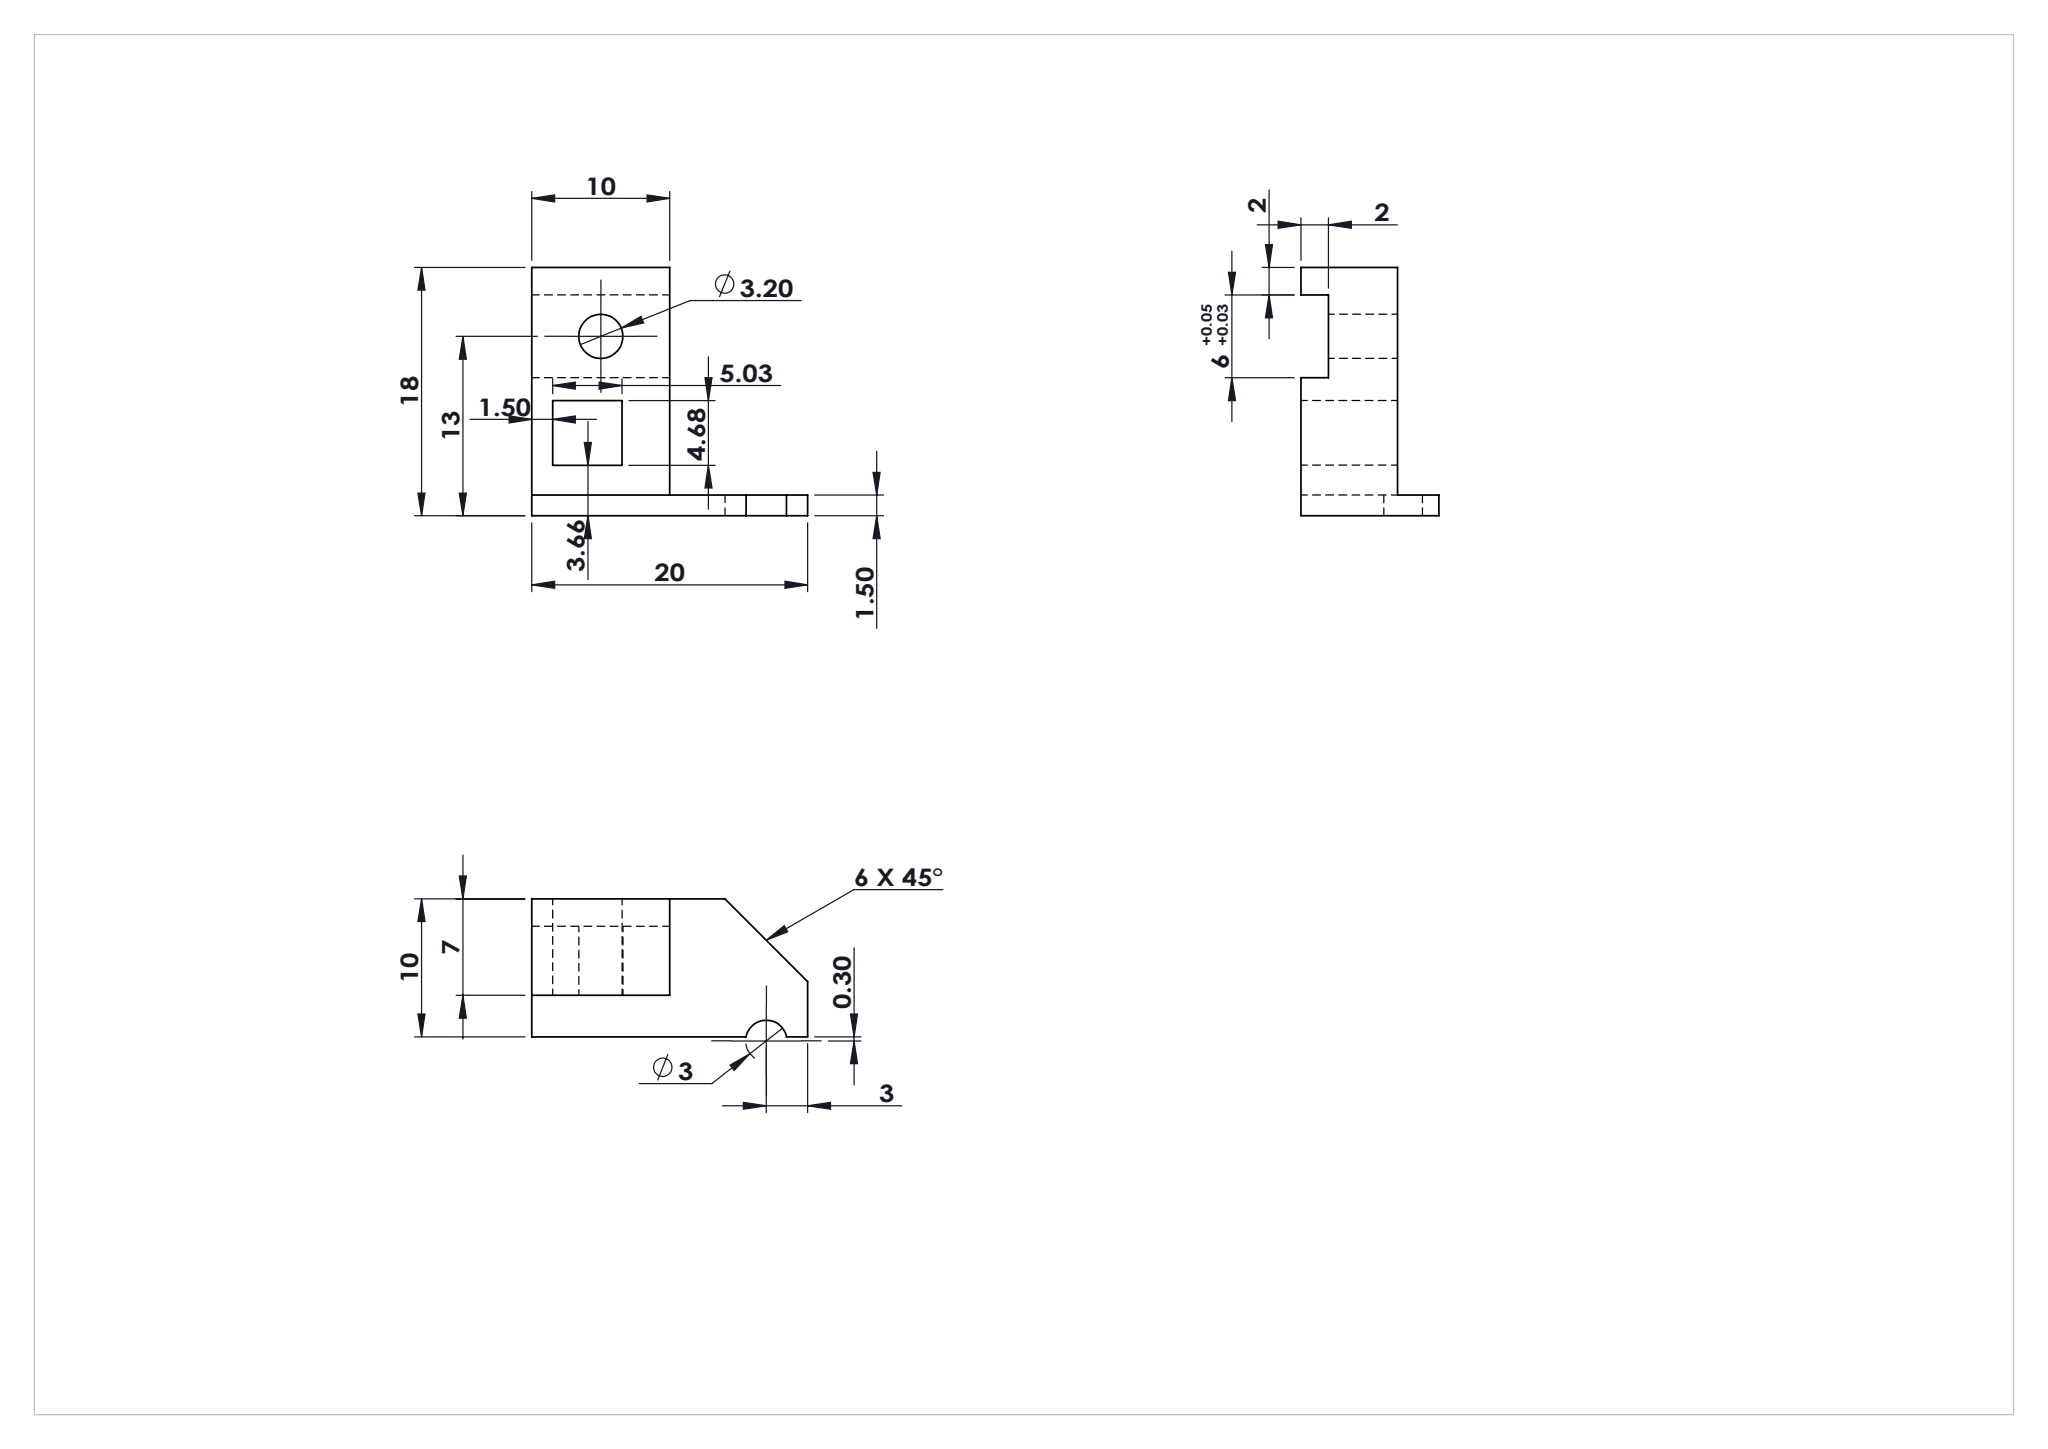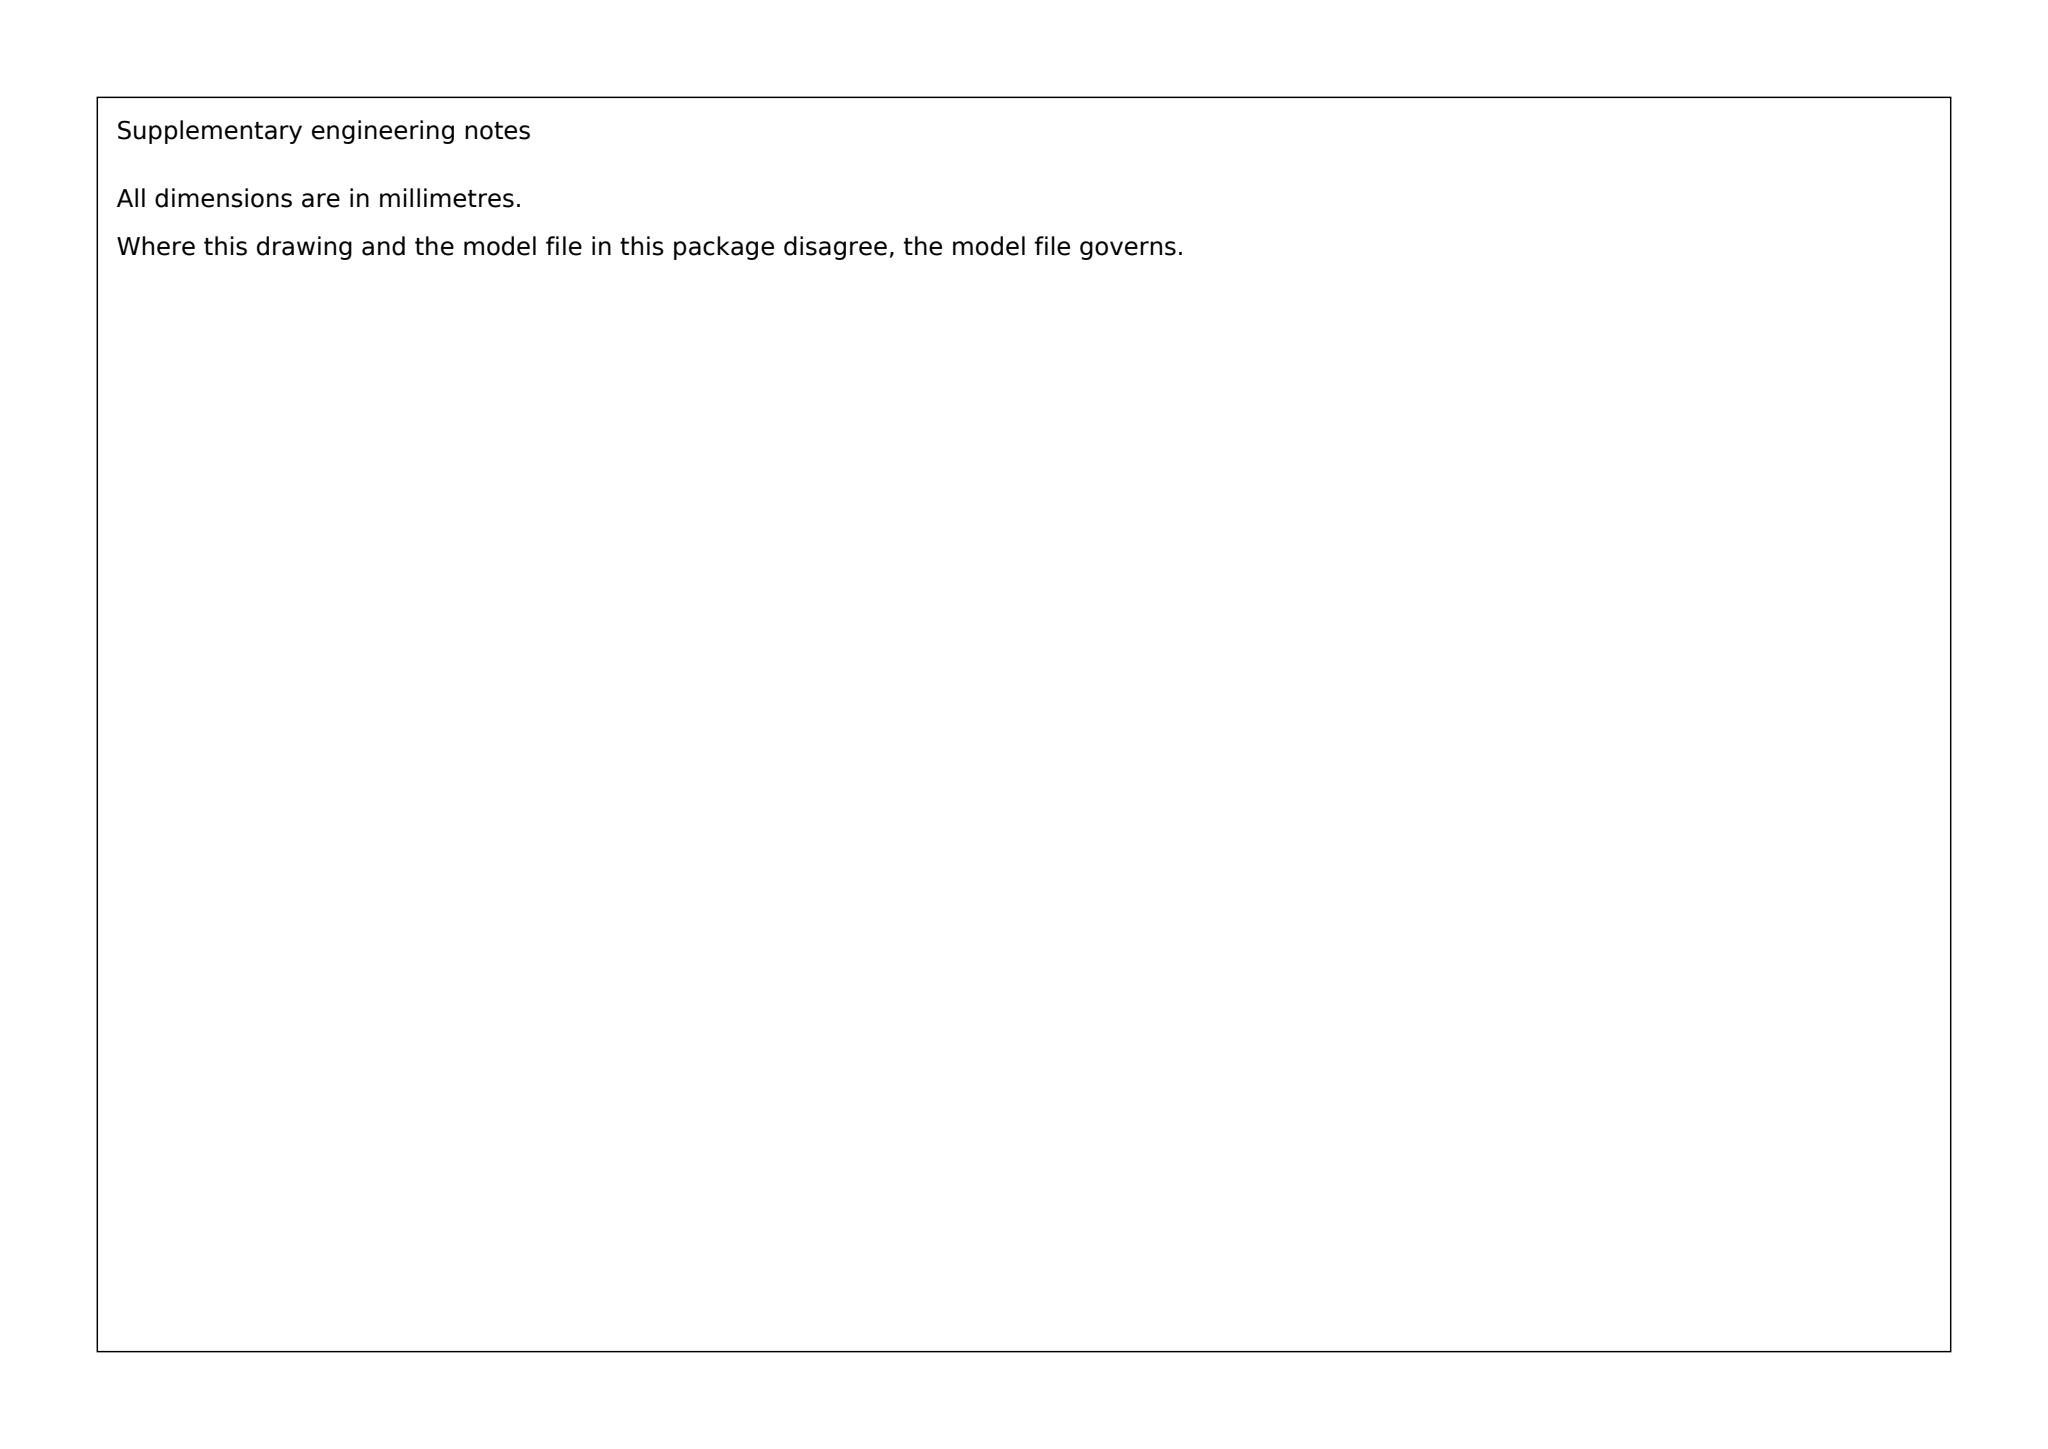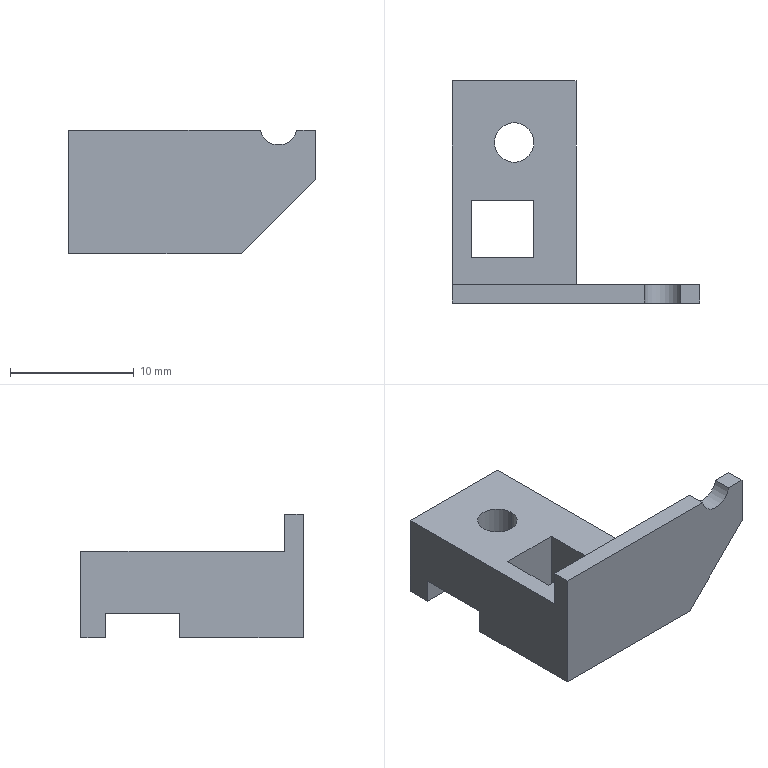Part | SolidWorks | mm | 1 solid | 22 faces | box 20 x 18 x 10 mm | volume 1099 mm3 | plane 19 | cylinder 3 | commonest cylinder face diameters 3.2 x2 3 x1
build123d program:
from build123d import *

# Parameters (mm, degrees)
SKETCH1_W            = 10
SKETCH1_H            = 18
BOSS_EXTRUDE1_DEPTH  = 10
SKETCH3_W            = 3
SKETCH3_H            = 16.5
CUT_EXTRUDE2_DEPTH   = 17.763
SKETCH7_W            = 10
SKETCH7_H            = 6
CUT_EXTRUDE6_DEPTH   = 2
SKETCH8_W            = 10
SKETCH8_H            = 1.5
BOSS_EXTRUDE2_DEPTH  = 10
SKETCH9_R            = 1.5
CUT_EXTRUDE7_DEPTH   = 25.439
CHAMFER1_SIZE        = 6
SKETCH2_R            = 1.6
CUT_EXTRUDE1_DEPTH   = 20.235
SKETCH3_2_W          = 5.032
SKETCH3_2_H          = 4.682
CUT_EXTRUDE2_2_DEPTH = 10


with BuildPart() as part:
    # Sketch1 → Boss-Extrude1 (new body)
    with BuildSketch(Plane.XY):
        Rectangle(SKETCH1_W, SKETCH1_H)
    extrude(amount=-BOSS_EXTRUDE1_DEPTH)

    # Sketch3 → Cut-Extrude2 (cut, through all)
    with BuildSketch(Plane(origin=(5, 0, 0), x_dir=(0, 0, -1), z_dir=(1, 0, 0))):
        with Locations((1.5, 0.75)):
            Rectangle(SKETCH3_W, SKETCH3_H)
    extrude(amount=-CUT_EXTRUDE2_DEPTH, mode=Mode.SUBTRACT)

    # Sketch7 → Cut-Extrude6 (cut)
    with BuildSketch(Plane(origin=(0, 0, -10), x_dir=(-1, 0, 0), z_dir=(0, 0, -1))):
        with Locations((0, 4)):
            Rectangle(SKETCH7_W, SKETCH7_H)
    extrude(amount=-CUT_EXTRUDE6_DEPTH, mode=Mode.SUBTRACT)

    # Sketch8 → Boss-Extrude2 (add)
    with BuildSketch(Plane.XY):
        with Locations((10, -8.25)):
            Rectangle(SKETCH8_W, SKETCH8_H)
    extrude(amount=-BOSS_EXTRUDE2_DEPTH)

    # Sketch9 → Cut-Extrude7 (cut, through all)
    with BuildSketch(Plane(origin=(0, -7.5, 0), x_dir=(1, 0, 0), z_dir=(0, 1, 0))):
        with Locations((12, -0.3)):
            Circle(SKETCH9_R)
    extrude(amount=-CUT_EXTRUDE7_DEPTH, mode=Mode.SUBTRACT)

    # Chamfer1
    chamfer1_edges = [part.edges().sort_by_distance(p)[0] for p in [
        (15, -8.25, -10),
    ]]
    chamfer(chamfer1_edges, length=CHAMFER1_SIZE)

    # Sketch2 → Cut-Extrude1 (cut, through all)
    with BuildSketch(Plane(origin=(0, 0, -8), x_dir=(-1, 0, 0), z_dir=(0, 0, -1))):
        with Locations((0, 4)):
            Circle(SKETCH2_R)
    extrude(amount=-CUT_EXTRUDE1_DEPTH, mode=Mode.SUBTRACT)

    # Sketch3_2 → Cut-Extrude2_2 (cut)
    with BuildSketch(Plane(origin=(0, 0, -10), x_dir=(-1, 0, 0), z_dir=(0, 0, -1))):
        with Locations((0.9812, -2.995)):
            Rectangle(SKETCH3_2_W, SKETCH3_2_H)
    extrude(amount=-CUT_EXTRUDE2_2_DEPTH, mode=Mode.SUBTRACT)


solid = part.part
STEP:
#1=CARTESIAN_POINT('',(1.6,4.,-3.));
#2=VERTEX_POINT('',#1);
#3=CARTESIAN_POINT('',(-1.6,4.,-3.));
#4=VERTEX_POINT('',#3);
#5=CARTESIAN_POINT('',(0.,4.,-3.));
#6=DIRECTION('',(0.,0.,-1.));
#7=DIRECTION('',(0.,1.,0.));
#8=AXIS2_PLACEMENT_3D('',#5,#6,#7);
#9=CIRCLE('',#8,1.6);
#10=EDGE_CURVE('',#2,#4,#9,.T.);
#11=ORIENTED_EDGE('',*,*,#10,.F.);
#12=CARTESIAN_POINT('',(1.6,4.,-8.));
#13=VERTEX_POINT('',#12);
#14=CARTESIAN_POINT('',(1.6,4.,0.));
#15=DIRECTION('',(0.,0.,-1.));
#16=VECTOR('',#15,1000.);
#17=LINE('',#14,#16);
#18=EDGE_CURVE('',#2,#13,#17,.T.);
#19=ORIENTED_EDGE('',*,*,#18,.T.);
#20=CARTESIAN_POINT('',(-1.6,4.,-8.));
#21=VERTEX_POINT('',#20);
#22=CARTESIAN_POINT('',(0.,4.,-8.));
#23=DIRECTION('',(0.,0.,-1.));
#24=DIRECTION('',(-1.,0.,0.));
#25=AXIS2_PLACEMENT_3D('',#22,#23,#24);
#26=CIRCLE('',#25,1.6);
#27=EDGE_CURVE('',#13,#21,#26,.T.);
#28=ORIENTED_EDGE('',*,*,#27,.T.);
#29=CARTESIAN_POINT('',(-1.6,4.,0.));
#30=DIRECTION('',(0.,0.,-1.));
#31=VECTOR('',#30,1000.);
#32=LINE('',#29,#31);
#33=EDGE_CURVE('',#4,#21,#32,.T.);
#34=ORIENTED_EDGE('',*,*,#33,.F.);
#35=EDGE_LOOP('',(#11,#19,#28,#34));
#36=FACE_OUTER_BOUND('',#35,.T.);
#37=CARTESIAN_POINT('',(0.,4.,0.));
#38=DIRECTION('',(0.,0.,-1.));
#39=DIRECTION('',(-1.,0.,0.));
#40=AXIS2_PLACEMENT_3D('',#37,#38,#39);
#41=CYLINDRICAL_SURFACE('',#40,1.6);
#42=ADVANCED_FACE('',(#36),#41,.F.);
#43=CARTESIAN_POINT('',(13.47,-9.,0.));
#44=VERTEX_POINT('',#43);
#45=CARTESIAN_POINT('',(13.47,-7.5,-0.));
#46=VERTEX_POINT('',#45);
#47=CARTESIAN_POINT('',(13.47,-9.,0.));
#48=DIRECTION('',(0.,1.,0.));
#49=VECTOR('',#48,1000.);
#50=LINE('',#47,#49);
#51=EDGE_CURVE('',#44,#46,#50,.T.);
#52=ORIENTED_EDGE('',*,*,#51,.F.);
#53=CARTESIAN_POINT('',(15.,-9.,0.));
#54=VERTEX_POINT('',#53);
#55=CARTESIAN_POINT('',(5.,-9.,0.));
#56=DIRECTION('',(1.,0.,0.));
#57=VECTOR('',#56,1000.);
#58=LINE('',#55,#57);
#59=EDGE_CURVE('',#44,#54,#58,.T.);
#60=ORIENTED_EDGE('',*,*,#59,.T.);
#61=CARTESIAN_POINT('',(15.,-7.5,0.));
#62=VERTEX_POINT('',#61);
#63=CARTESIAN_POINT('',(15.,-9.,0.));
#64=DIRECTION('',(0.,1.,0.));
#65=VECTOR('',#64,1000.);
#66=LINE('',#63,#65);
#67=EDGE_CURVE('',#54,#62,#66,.T.);
#68=ORIENTED_EDGE('',*,*,#67,.T.);
#69=CARTESIAN_POINT('',(-5.,-7.5,-0.));
#70=DIRECTION('',(1.,0.,0.));
#71=VECTOR('',#70,1000.);
#72=LINE('',#69,#71);
#73=EDGE_CURVE('',#46,#62,#72,.T.);
#74=ORIENTED_EDGE('',*,*,#73,.F.);
#75=EDGE_LOOP('',(#52,#60,#68,#74));
#76=FACE_OUTER_BOUND('',#75,.T.);
#77=CARTESIAN_POINT('',(0.,0.,0.));
#78=DIRECTION('',(0.,0.,1.));
#79=DIRECTION('',(1.,0.,0.));
#80=AXIS2_PLACEMENT_3D('',#77,#78,#79);
#81=PLANE('',#80);
#82=ADVANCED_FACE('',(#76),#81,.T.);
#83=CARTESIAN_POINT('',(5.,7.,-10.));
#84=VERTEX_POINT('',#83);
#85=CARTESIAN_POINT('',(5.,9.,-10.));
#86=VERTEX_POINT('',#85);
#87=CARTESIAN_POINT('',(5.,-9.,-10.));
#88=DIRECTION('',(0.,1.,0.));
#89=VECTOR('',#88,1000.);
#90=LINE('',#87,#89);
#91=EDGE_CURVE('',#84,#86,#90,.T.);
#92=ORIENTED_EDGE('',*,*,#91,.F.);
#93=CARTESIAN_POINT('',(-5.,7.,-10.));
#94=VERTEX_POINT('',#93);
#95=CARTESIAN_POINT('',(5.,7.,-10.));
#96=DIRECTION('',(1.,0.,0.));
#97=VECTOR('',#96,1000.);
#98=LINE('',#95,#97);
#99=EDGE_CURVE('',#94,#84,#98,.T.);
#100=ORIENTED_EDGE('',*,*,#99,.F.);
#101=CARTESIAN_POINT('',(-5.,9.,-10.));
#102=VERTEX_POINT('',#101);
#103=CARTESIAN_POINT('',(-5.,-9.,-10.));
#104=DIRECTION('',(0.,-1.,0.));
#105=VECTOR('',#104,1000.);
#106=LINE('',#103,#105);
#107=EDGE_CURVE('',#102,#94,#106,.T.);
#108=ORIENTED_EDGE('',*,*,#107,.F.);
#109=CARTESIAN_POINT('',(5.,9.,-10.));
#110=DIRECTION('',(-1.,0.,0.));
#111=VECTOR('',#110,1000.);
#112=LINE('',#109,#111);
#113=EDGE_CURVE('',#86,#102,#112,.T.);
#114=ORIENTED_EDGE('',*,*,#113,.F.);
#115=EDGE_LOOP('',(#92,#100,#108,#114));
#116=FACE_OUTER_BOUND('',#115,.T.);
#117=CARTESIAN_POINT('',(0.,0.,-10.));
#118=DIRECTION('',(0.,0.,1.));
#119=DIRECTION('',(1.,0.,0.));
#120=AXIS2_PLACEMENT_3D('',#117,#118,#119);
#121=PLANE('',#120);
#122=ADVANCED_FACE('',(#116),#121,.F.);
#123=CARTESIAN_POINT('',(-5.,7.,-8.));
#124=VERTEX_POINT('',#123);
#125=CARTESIAN_POINT('',(-5.,7.,-8.));
#126=DIRECTION('',(0.,0.,-1.));
#127=VECTOR('',#126,1000.);
#128=LINE('',#125,#127);
#129=EDGE_CURVE('',#124,#94,#128,.T.);
#130=ORIENTED_EDGE('',*,*,#129,.F.);
#131=CARTESIAN_POINT('',(-5.,1.,-8.));
#132=VERTEX_POINT('',#131);
#133=CARTESIAN_POINT('',(-5.,7.,-8.));
#134=DIRECTION('',(0.,1.,0.));
#135=VECTOR('',#134,1000.);
#136=LINE('',#133,#135);
#137=EDGE_CURVE('',#132,#124,#136,.T.);
#138=ORIENTED_EDGE('',*,*,#137,.F.);
#139=CARTESIAN_POINT('',(-5.,1.,-10.));
#140=VERTEX_POINT('',#139);
#141=CARTESIAN_POINT('',(-5.,1.,-8.));
#142=DIRECTION('',(0.,0.,-1.));
#143=VECTOR('',#142,1000.);
#144=LINE('',#141,#143);
#145=EDGE_CURVE('',#132,#140,#144,.T.);
#146=ORIENTED_EDGE('',*,*,#145,.T.);
#147=CARTESIAN_POINT('',(-5.,-9.,-10.));
#148=VERTEX_POINT('',#147);
#149=CARTESIAN_POINT('',(-5.,-9.,-10.));
#150=DIRECTION('',(0.,-1.,0.));
#151=VECTOR('',#150,1000.);
#152=LINE('',#149,#151);
#153=EDGE_CURVE('',#140,#148,#152,.T.);
#154=ORIENTED_EDGE('',*,*,#153,.T.);
#155=CARTESIAN_POINT('',(-5.,-9.,0.));
#156=VERTEX_POINT('',#155);
#157=CARTESIAN_POINT('',(-5.,-9.,-10.));
#158=DIRECTION('',(0.,0.,1.));
#159=VECTOR('',#158,1000.);
#160=LINE('',#157,#159);
#161=EDGE_CURVE('',#148,#156,#160,.T.);
#162=ORIENTED_EDGE('',*,*,#161,.T.);
#163=CARTESIAN_POINT('',(-5.,-7.5,0.));
#164=VERTEX_POINT('',#163);
#165=CARTESIAN_POINT('',(-5.,-9.,0.));
#166=DIRECTION('',(0.,-1.,0.));
#167=VECTOR('',#166,1000.);
#168=LINE('',#165,#167);
#169=EDGE_CURVE('',#164,#156,#168,.T.);
#170=ORIENTED_EDGE('',*,*,#169,.F.);
#171=CARTESIAN_POINT('',(-5.,-7.5,-3.));
#172=VERTEX_POINT('',#171);
#173=CARTESIAN_POINT('',(-5.,-7.5,-0.));
#174=DIRECTION('',(0.,0.,-1.));
#175=VECTOR('',#174,1000.);
#176=LINE('',#173,#175);
#177=EDGE_CURVE('',#164,#172,#176,.T.);
#178=ORIENTED_EDGE('',*,*,#177,.T.);
#179=CARTESIAN_POINT('',(-5.,9.,-3.));
#180=VERTEX_POINT('',#179);
#181=CARTESIAN_POINT('',(-5.,9.,-3.));
#182=DIRECTION('',(0.,1.,0.));
#183=VECTOR('',#182,1000.);
#184=LINE('',#181,#183);
#185=EDGE_CURVE('',#172,#180,#184,.T.);
#186=ORIENTED_EDGE('',*,*,#185,.T.);
#187=CARTESIAN_POINT('',(-5.,9.,-10.));
#188=DIRECTION('',(0.,0.,1.));
#189=VECTOR('',#188,1000.);
#190=LINE('',#187,#189);
#191=EDGE_CURVE('',#102,#180,#190,.T.);
#192=ORIENTED_EDGE('',*,*,#191,.F.);
#193=ORIENTED_EDGE('',*,*,#107,.T.);
#194=EDGE_LOOP('',(#130,#138,#146,#154,#162,#170,#178,#186,#192,#193));
#195=FACE_OUTER_BOUND('',#194,.T.);
#196=CARTESIAN_POINT('',(-5.,-9.,-10.));
#197=DIRECTION('',(-1.,0.,0.));
#198=DIRECTION('',(0.,0.,1.));
#199=AXIS2_PLACEMENT_3D('',#196,#197,#198);
#200=PLANE('',#199);
#201=ADVANCED_FACE('',(#195),#200,.T.);
#202=CARTESIAN_POINT('',(5.,9.,-3.));
#203=VERTEX_POINT('',#202);
#204=CARTESIAN_POINT('',(-5.,9.,-3.));
#205=DIRECTION('',(1.,0.,0.));
#206=VECTOR('',#205,1000.);
#207=LINE('',#204,#206);
#208=EDGE_CURVE('',#180,#203,#207,.T.);
#209=ORIENTED_EDGE('',*,*,#208,.T.);
#210=CARTESIAN_POINT('',(5.,9.,-10.));
#211=DIRECTION('',(0.,0.,1.));
#212=VECTOR('',#211,1000.);
#213=LINE('',#210,#212);
#214=EDGE_CURVE('',#86,#203,#213,.T.);
#215=ORIENTED_EDGE('',*,*,#214,.F.);
#216=ORIENTED_EDGE('',*,*,#113,.T.);
#217=ORIENTED_EDGE('',*,*,#191,.T.);
#218=EDGE_LOOP('',(#209,#215,#216,#217));
#219=FACE_OUTER_BOUND('',#218,.T.);
#220=CARTESIAN_POINT('',(5.,9.,-10.));
#221=DIRECTION('',(0.,1.,0.));
#222=DIRECTION('',(0.,0.,1.));
#223=AXIS2_PLACEMENT_3D('',#220,#221,#222);
#224=PLANE('',#223);
#225=ADVANCED_FACE('',(#219),#224,.T.);
#226=CARTESIAN_POINT('',(5.,-7.5,-10.));
#227=VERTEX_POINT('',#226);
#228=CARTESIAN_POINT('',(5.,-7.5,-3.));
#229=VERTEX_POINT('',#228);
#230=CARTESIAN_POINT('',(5.,-7.5,-20.112));
#231=DIRECTION('',(0.,0.,1.));
#232=VECTOR('',#231,1000.);
#233=LINE('',#230,#232);
#234=EDGE_CURVE('',#227,#229,#233,.T.);
#235=ORIENTED_EDGE('',*,*,#234,.F.);
#236=CARTESIAN_POINT('',(5.,1.,-10.));
#237=VERTEX_POINT('',#236);
#238=CARTESIAN_POINT('',(5.,-9.,-10.));
#239=DIRECTION('',(0.,1.,0.));
#240=VECTOR('',#239,1000.);
#241=LINE('',#238,#240);
#242=EDGE_CURVE('',#227,#237,#241,.T.);
#243=ORIENTED_EDGE('',*,*,#242,.T.);
#244=CARTESIAN_POINT('',(5.,1.,-8.));
#245=VERTEX_POINT('',#244);
#246=CARTESIAN_POINT('',(5.,1.,-8.));
#247=DIRECTION('',(0.,0.,-1.));
#248=VECTOR('',#247,1000.);
#249=LINE('',#246,#248);
#250=EDGE_CURVE('',#245,#237,#249,.T.);
#251=ORIENTED_EDGE('',*,*,#250,.F.);
#252=CARTESIAN_POINT('',(5.,7.,-8.));
#253=VERTEX_POINT('',#252);
#254=CARTESIAN_POINT('',(5.,7.,-8.));
#255=DIRECTION('',(-0.,-1.,0.));
#256=VECTOR('',#255,1000.);
#257=LINE('',#254,#256);
#258=EDGE_CURVE('',#253,#245,#257,.T.);
#259=ORIENTED_EDGE('',*,*,#258,.F.);
#260=CARTESIAN_POINT('',(5.,7.,-8.));
#261=DIRECTION('',(0.,0.,-1.));
#262=VECTOR('',#261,1000.);
#263=LINE('',#260,#262);
#264=EDGE_CURVE('',#253,#84,#263,.T.);
#265=ORIENTED_EDGE('',*,*,#264,.T.);
#266=ORIENTED_EDGE('',*,*,#91,.T.);
#267=ORIENTED_EDGE('',*,*,#214,.T.);
#268=CARTESIAN_POINT('',(5.,9.,-3.));
#269=DIRECTION('',(0.,1.,0.));
#270=VECTOR('',#269,1000.);
#271=LINE('',#268,#270);
#272=EDGE_CURVE('',#229,#203,#271,.T.);
#273=ORIENTED_EDGE('',*,*,#272,.F.);
#274=EDGE_LOOP('',(#235,#243,#251,#259,#265,#266,#267,#273));
#275=FACE_OUTER_BOUND('',#274,.T.);
#276=CARTESIAN_POINT('',(5.,-9.,-10.));
#277=DIRECTION('',(1.,0.,0.));
#278=DIRECTION('',(0.,0.,-1.));
#279=AXIS2_PLACEMENT_3D('',#276,#277,#278);
#280=PLANE('',#279);
#281=ADVANCED_FACE('',(#275),#280,.T.);
#282=CARTESIAN_POINT('',(9.,-9.,-10.));
#283=VERTEX_POINT('',#282);
#284=CARTESIAN_POINT('',(5.,-9.,-10.));
#285=DIRECTION('',(1.,0.,0.));
#286=VECTOR('',#285,1000.);
#287=LINE('',#284,#286);
#288=EDGE_CURVE('',#148,#283,#287,.T.);
#289=ORIENTED_EDGE('',*,*,#288,.T.);
#290=CARTESIAN_POINT('',(15.,-9.,-4.));
#291=VERTEX_POINT('',#290);
#292=CARTESIAN_POINT('',(7.,-9.,-12.));
#293=DIRECTION('',(0.7071,0.,0.7071));
#294=VECTOR('',#293,1000.);
#295=LINE('',#292,#294);
#296=EDGE_CURVE('',#283,#291,#295,.T.);
#297=ORIENTED_EDGE('',*,*,#296,.T.);
#298=CARTESIAN_POINT('',(15.,-9.,-20.112));
#299=DIRECTION('',(0.,0.,1.));
#300=VECTOR('',#299,1000.);
#301=LINE('',#298,#300);
#302=EDGE_CURVE('',#291,#54,#301,.T.);
#303=ORIENTED_EDGE('',*,*,#302,.T.);
#304=ORIENTED_EDGE('',*,*,#59,.F.);
#305=CARTESIAN_POINT('',(10.53,-9.,0.));
#306=VERTEX_POINT('',#305);
#307=CARTESIAN_POINT('',(12.,-9.,0.3));
#308=DIRECTION('',(0.,1.,0.));
#309=DIRECTION('',(0.,0.,1.));
#310=AXIS2_PLACEMENT_3D('',#307,#308,#309);
#311=CIRCLE('',#310,1.5);
#312=EDGE_CURVE('',#44,#306,#311,.T.);
#313=ORIENTED_EDGE('',*,*,#312,.T.);
#314=CARTESIAN_POINT('',(5.,-9.,0.));
#315=DIRECTION('',(1.,0.,0.));
#316=VECTOR('',#315,1000.);
#317=LINE('',#314,#316);
#318=EDGE_CURVE('',#156,#306,#317,.T.);
#319=ORIENTED_EDGE('',*,*,#318,.F.);
#320=ORIENTED_EDGE('',*,*,#161,.F.);
#321=EDGE_LOOP('',(#289,#297,#303,#304,#313,#319,#320));
#322=FACE_OUTER_BOUND('',#321,.T.);
#323=CARTESIAN_POINT('',(5.,-9.,-10.));
#324=DIRECTION('',(0.,-1.,0.));
#325=DIRECTION('',(0.,0.,-1.));
#326=AXIS2_PLACEMENT_3D('',#323,#324,#325);
#327=PLANE('',#326);
#328=ADVANCED_FACE('',(#322),#327,.T.);
#329=CARTESIAN_POINT('',(1.535,-5.336,-10.));
#330=VERTEX_POINT('',#329);
#331=CARTESIAN_POINT('',(-3.497,-5.336,-10.));
#332=VERTEX_POINT('',#331);
#333=CARTESIAN_POINT('',(1.535,-5.336,-10.));
#334=DIRECTION('',(-1.,0.,0.));
#335=VECTOR('',#334,1000.);
#336=LINE('',#333,#335);
#337=EDGE_CURVE('',#330,#332,#336,.T.);
#338=ORIENTED_EDGE('',*,*,#337,.F.);
#339=CARTESIAN_POINT('',(1.535,-0.6543,-10.));
#340=VERTEX_POINT('',#339);
#341=CARTESIAN_POINT('',(1.535,-0.6543,-10.));
#342=DIRECTION('',(0.,-1.,0.));
#343=VECTOR('',#342,1000.);
#344=LINE('',#341,#343);
#345=EDGE_CURVE('',#340,#330,#344,.T.);
#346=ORIENTED_EDGE('',*,*,#345,.F.);
#347=CARTESIAN_POINT('',(-3.497,-0.6543,-10.));
#348=VERTEX_POINT('',#347);
#349=CARTESIAN_POINT('',(1.535,-0.6543,-10.));
#350=DIRECTION('',(1.,0.,0.));
#351=VECTOR('',#350,1000.);
#352=LINE('',#349,#351);
#353=EDGE_CURVE('',#348,#340,#352,.T.);
#354=ORIENTED_EDGE('',*,*,#353,.F.);
#355=CARTESIAN_POINT('',(-3.497,-0.6543,-10.));
#356=DIRECTION('',(0.,1.,0.));
#357=VECTOR('',#356,1000.);
#358=LINE('',#355,#357);
#359=EDGE_CURVE('',#332,#348,#358,.T.);
#360=ORIENTED_EDGE('',*,*,#359,.F.);
#361=EDGE_LOOP('',(#338,#346,#354,#360));
#362=FACE_BOUND('',#361,.T.);
#363=CARTESIAN_POINT('',(9.,-7.5,-10.));
#364=VERTEX_POINT('',#363);
#365=CARTESIAN_POINT('',(5.,-7.5,-10.));
#366=DIRECTION('',(1.,0.,0.));
#367=VECTOR('',#366,1000.);
#368=LINE('',#365,#367);
#369=EDGE_CURVE('',#227,#364,#368,.T.);
#370=ORIENTED_EDGE('',*,*,#369,.T.);
#371=CARTESIAN_POINT('',(9.,-9.,-10.));
#372=DIRECTION('',(0.,-1.,0.));
#373=VECTOR('',#372,1000.);
#374=LINE('',#371,#373);
#375=EDGE_CURVE('',#364,#283,#374,.T.);
#376=ORIENTED_EDGE('',*,*,#375,.T.);
#377=ORIENTED_EDGE('',*,*,#288,.F.);
#378=ORIENTED_EDGE('',*,*,#153,.F.);
#379=CARTESIAN_POINT('',(5.,1.,-10.));
#380=DIRECTION('',(-1.,0.,0.));
#381=VECTOR('',#380,1000.);
#382=LINE('',#379,#381);
#383=EDGE_CURVE('',#237,#140,#382,.T.);
#384=ORIENTED_EDGE('',*,*,#383,.F.);
#385=ORIENTED_EDGE('',*,*,#242,.F.);
#386=EDGE_LOOP('',(#370,#376,#377,#378,#384,#385));
#387=FACE_OUTER_BOUND('',#386,.T.);
#388=CARTESIAN_POINT('',(0.,0.,-10.));
#389=DIRECTION('',(0.,0.,1.));
#390=DIRECTION('',(1.,0.,0.));
#391=AXIS2_PLACEMENT_3D('',#388,#389,#390);
#392=PLANE('',#391);
#393=ADVANCED_FACE('',(#362,#387),#392,.F.);
#394=CARTESIAN_POINT('',(10.53,-7.5,-0.));
#395=VERTEX_POINT('',#394);
#396=CARTESIAN_POINT('',(10.53,-9.,0.));
#397=DIRECTION('',(0.,-1.,0.));
#398=VECTOR('',#397,1000.);
#399=LINE('',#396,#398);
#400=EDGE_CURVE('',#395,#306,#399,.T.);
#401=ORIENTED_EDGE('',*,*,#400,.F.);
#402=CARTESIAN_POINT('',(-5.,-7.5,-0.));
#403=DIRECTION('',(1.,0.,0.));
#404=VECTOR('',#403,1000.);
#405=LINE('',#402,#404);
#406=EDGE_CURVE('',#164,#395,#405,.T.);
#407=ORIENTED_EDGE('',*,*,#406,.F.);
#408=ORIENTED_EDGE('',*,*,#169,.T.);
#409=ORIENTED_EDGE('',*,*,#318,.T.);
#410=EDGE_LOOP('',(#401,#407,#408,#409));
#411=FACE_OUTER_BOUND('',#410,.T.);
#412=CARTESIAN_POINT('',(0.,0.,0.));
#413=DIRECTION('',(0.,0.,1.));
#414=DIRECTION('',(1.,0.,0.));
#415=AXIS2_PLACEMENT_3D('',#412,#413,#414);
#416=PLANE('',#415);
#417=ADVANCED_FACE('',(#411),#416,.T.);
#418=CARTESIAN_POINT('',(-3.497,-0.6543,-3.));
#419=VERTEX_POINT('',#418);
#420=CARTESIAN_POINT('',(1.535,-0.6543,-3.));
#421=VERTEX_POINT('',#420);
#422=CARTESIAN_POINT('',(-5.,-0.6543,-3.));
#423=DIRECTION('',(1.,0.,0.));
#424=VECTOR('',#423,1000.);
#425=LINE('',#422,#424);
#426=EDGE_CURVE('',#419,#421,#425,.T.);
#427=ORIENTED_EDGE('',*,*,#426,.T.);
#428=CARTESIAN_POINT('',(1.535,-5.336,-3.));
#429=VERTEX_POINT('',#428);
#430=CARTESIAN_POINT('',(1.535,9.,-3.));
#431=DIRECTION('',(0.,-1.,-0.));
#432=VECTOR('',#431,1000.);
#433=LINE('',#430,#432);
#434=EDGE_CURVE('',#421,#429,#433,.T.);
#435=ORIENTED_EDGE('',*,*,#434,.T.);
#436=CARTESIAN_POINT('',(-3.497,-5.336,-3.));
#437=VERTEX_POINT('',#436);
#438=CARTESIAN_POINT('',(-5.,-5.336,-3.));
#439=DIRECTION('',(-1.,0.,0.));
#440=VECTOR('',#439,1000.);
#441=LINE('',#438,#440);
#442=EDGE_CURVE('',#429,#437,#441,.T.);
#443=ORIENTED_EDGE('',*,*,#442,.T.);
#444=CARTESIAN_POINT('',(-3.497,9.,-3.));
#445=DIRECTION('',(0.,1.,0.));
#446=VECTOR('',#445,1000.);
#447=LINE('',#444,#446);
#448=EDGE_CURVE('',#437,#419,#447,.T.);
#449=ORIENTED_EDGE('',*,*,#448,.T.);
#450=EDGE_LOOP('',(#427,#435,#443,#449));
#451=FACE_BOUND('',#450,.T.);
#452=CARTESIAN_POINT('',(0.,4.,-3.));
#453=DIRECTION('',(0.,0.,-1.));
#454=DIRECTION('',(0.,1.,0.));
#455=AXIS2_PLACEMENT_3D('',#452,#453,#454);
#456=CIRCLE('',#455,1.6);
#457=EDGE_CURVE('',#4,#2,#456,.T.);
#458=ORIENTED_EDGE('',*,*,#457,.T.);
#459=ORIENTED_EDGE('',*,*,#10,.T.);
#460=EDGE_LOOP('',(#458,#459));
#461=FACE_BOUND('',#460,.T.);
#462=ORIENTED_EDGE('',*,*,#272,.T.);
#463=ORIENTED_EDGE('',*,*,#208,.F.);
#464=ORIENTED_EDGE('',*,*,#185,.F.);
#465=CARTESIAN_POINT('',(-5.,-7.5,-3.));
#466=DIRECTION('',(1.,0.,0.));
#467=VECTOR('',#466,1000.);
#468=LINE('',#465,#467);
#469=EDGE_CURVE('',#172,#229,#468,.T.);
#470=ORIENTED_EDGE('',*,*,#469,.T.);
#471=EDGE_LOOP('',(#462,#463,#464,#470));
#472=FACE_OUTER_BOUND('',#471,.T.);
#473=CARTESIAN_POINT('',(-5.,9.,-3.));
#474=DIRECTION('',(0.,0.,-1.));
#475=DIRECTION('',(0.,1.,0.));
#476=AXIS2_PLACEMENT_3D('',#473,#474,#475);
#477=PLANE('',#476);
#478=ADVANCED_FACE('',(#451,#461,#472),#477,.F.);
#479=CARTESIAN_POINT('',(15.,-7.5,-4.));
#480=VERTEX_POINT('',#479);
#481=CARTESIAN_POINT('',(15.,-7.5,-20.112));
#482=DIRECTION('',(0.,0.,1.));
#483=VECTOR('',#482,1000.);
#484=LINE('',#481,#483);
#485=EDGE_CURVE('',#480,#62,#484,.T.);
#486=ORIENTED_EDGE('',*,*,#485,.F.);
#487=CARTESIAN_POINT('',(9.,-7.5,-10.));
#488=DIRECTION('',(-0.7071,0.,-0.7071));
#489=VECTOR('',#488,1000.);
#490=LINE('',#487,#489);
#491=EDGE_CURVE('',#480,#364,#490,.T.);
#492=ORIENTED_EDGE('',*,*,#491,.T.);
#493=ORIENTED_EDGE('',*,*,#369,.F.);
#494=ORIENTED_EDGE('',*,*,#234,.T.);
#495=ORIENTED_EDGE('',*,*,#469,.F.);
#496=ORIENTED_EDGE('',*,*,#177,.F.);
#497=ORIENTED_EDGE('',*,*,#406,.T.);
#498=CARTESIAN_POINT('',(12.,-7.5,0.3));
#499=DIRECTION('',(0.,1.,0.));
#500=DIRECTION('',(0.,0.,1.));
#501=AXIS2_PLACEMENT_3D('',#498,#499,#500);
#502=CIRCLE('',#501,1.5);
#503=EDGE_CURVE('',#46,#395,#502,.T.);
#504=ORIENTED_EDGE('',*,*,#503,.F.);
#505=ORIENTED_EDGE('',*,*,#73,.T.);
#506=EDGE_LOOP('',(#486,#492,#493,#494,#495,#496,#497,#504,#505));
#507=FACE_OUTER_BOUND('',#506,.T.);
#508=CARTESIAN_POINT('',(-5.,-7.5,-0.));
#509=DIRECTION('',(0.,-1.,0.));
#510=DIRECTION('',(0.,0.,-1.));
#511=AXIS2_PLACEMENT_3D('',#508,#509,#510);
#512=PLANE('',#511);
#513=ADVANCED_FACE('',(#507),#512,.F.);
#514=ORIENTED_EDGE('',*,*,#99,.T.);
#515=ORIENTED_EDGE('',*,*,#264,.F.);
#516=CARTESIAN_POINT('',(5.,7.,-8.));
#517=DIRECTION('',(1.,0.,0.));
#518=VECTOR('',#517,1000.);
#519=LINE('',#516,#518);
#520=EDGE_CURVE('',#124,#253,#519,.T.);
#521=ORIENTED_EDGE('',*,*,#520,.F.);
#522=ORIENTED_EDGE('',*,*,#129,.T.);
#523=EDGE_LOOP('',(#514,#515,#521,#522));
#524=FACE_OUTER_BOUND('',#523,.T.);
#525=CARTESIAN_POINT('',(5.,7.,-8.));
#526=DIRECTION('',(-0.,1.,0.));
#527=DIRECTION('',(-1.,-0.,0.));
#528=AXIS2_PLACEMENT_3D('',#525,#526,#527);
#529=PLANE('',#528);
#530=ADVANCED_FACE('',(#524),#529,.F.);
#531=ORIENTED_EDGE('',*,*,#383,.T.);
#532=ORIENTED_EDGE('',*,*,#145,.F.);
#533=CARTESIAN_POINT('',(5.,1.,-8.));
#534=DIRECTION('',(-1.,0.,0.));
#535=VECTOR('',#534,1000.);
#536=LINE('',#533,#535);
#537=EDGE_CURVE('',#245,#132,#536,.T.);
#538=ORIENTED_EDGE('',*,*,#537,.F.);
#539=ORIENTED_EDGE('',*,*,#250,.T.);
#540=EDGE_LOOP('',(#531,#532,#538,#539));
#541=FACE_OUTER_BOUND('',#540,.T.);
#542=CARTESIAN_POINT('',(5.,1.,-8.));
#543=DIRECTION('',(0.,-1.,0.));
#544=DIRECTION('',(0.,0.,-1.));
#545=AXIS2_PLACEMENT_3D('',#542,#543,#544);
#546=PLANE('',#545);
#547=ADVANCED_FACE('',(#541),#546,.F.);
#548=CARTESIAN_POINT('',(0.,4.,-8.));
#549=DIRECTION('',(0.,0.,-1.));
#550=DIRECTION('',(-1.,0.,0.));
#551=AXIS2_PLACEMENT_3D('',#548,#549,#550);
#552=CIRCLE('',#551,1.6);
#553=EDGE_CURVE('',#21,#13,#552,.T.);
#554=ORIENTED_EDGE('',*,*,#553,.F.);
#555=ORIENTED_EDGE('',*,*,#27,.F.);
#556=EDGE_LOOP('',(#554,#555));
#557=FACE_BOUND('',#556,.T.);
#558=ORIENTED_EDGE('',*,*,#258,.T.);
#559=ORIENTED_EDGE('',*,*,#537,.T.);
#560=ORIENTED_EDGE('',*,*,#137,.T.);
#561=ORIENTED_EDGE('',*,*,#520,.T.);
#562=EDGE_LOOP('',(#558,#559,#560,#561));
#563=FACE_OUTER_BOUND('',#562,.T.);
#564=CARTESIAN_POINT('',(0.,0.,-8.));
#565=DIRECTION('',(0.,0.,-1.));
#566=DIRECTION('',(-1.,0.,0.));
#567=AXIS2_PLACEMENT_3D('',#564,#565,#566);
#568=PLANE('',#567);
#569=ADVANCED_FACE('',(#557,#563),#568,.T.);
#570=ORIENTED_EDGE('',*,*,#302,.F.);
#571=CARTESIAN_POINT('',(15.,-7.5,-4.));
#572=DIRECTION('',(0.,1.,0.));
#573=VECTOR('',#572,1000.);
#574=LINE('',#571,#573);
#575=EDGE_CURVE('',#291,#480,#574,.T.);
#576=ORIENTED_EDGE('',*,*,#575,.T.);
#577=ORIENTED_EDGE('',*,*,#485,.T.);
#578=ORIENTED_EDGE('',*,*,#67,.F.);
#579=EDGE_LOOP('',(#570,#576,#577,#578));
#580=FACE_OUTER_BOUND('',#579,.T.);
#581=CARTESIAN_POINT('',(15.,-9.,-20.112));
#582=DIRECTION('',(1.,0.,0.));
#583=DIRECTION('',(0.,0.,-1.));
#584=AXIS2_PLACEMENT_3D('',#581,#582,#583);
#585=PLANE('',#584);
#586=ADVANCED_FACE('',(#580),#585,.T.);
#587=ORIENTED_EDGE('',*,*,#51,.T.);
#588=ORIENTED_EDGE('',*,*,#503,.T.);
#589=ORIENTED_EDGE('',*,*,#400,.T.);
#590=ORIENTED_EDGE('',*,*,#312,.F.);
#591=EDGE_LOOP('',(#587,#588,#589,#590));
#592=FACE_OUTER_BOUND('',#591,.T.);
#593=CARTESIAN_POINT('',(12.,-9.,0.3));
#594=DIRECTION('',(0.,1.,0.));
#595=DIRECTION('',(0.,0.,1.));
#596=AXIS2_PLACEMENT_3D('',#593,#594,#595);
#597=CYLINDRICAL_SURFACE('',#596,1.5);
#598=ADVANCED_FACE('',(#592),#597,.F.);
#599=ORIENTED_EDGE('',*,*,#491,.F.);
#600=ORIENTED_EDGE('',*,*,#575,.F.);
#601=ORIENTED_EDGE('',*,*,#296,.F.);
#602=ORIENTED_EDGE('',*,*,#375,.F.);
#603=EDGE_LOOP('',(#599,#600,#601,#602));
#604=FACE_OUTER_BOUND('',#603,.T.);
#605=CARTESIAN_POINT('',(9.,0.,-10.));
#606=DIRECTION('',(0.7071,0.,-0.7071));
#607=DIRECTION('',(0.,1.,0.));
#608=AXIS2_PLACEMENT_3D('',#605,#606,#607);
#609=PLANE('',#608);
#610=ADVANCED_FACE('',(#604),#609,.T.);
#611=ORIENTED_EDGE('',*,*,#18,.F.);
#612=ORIENTED_EDGE('',*,*,#457,.F.);
#613=ORIENTED_EDGE('',*,*,#33,.T.);
#614=ORIENTED_EDGE('',*,*,#553,.T.);
#615=EDGE_LOOP('',(#611,#612,#613,#614));
#616=FACE_OUTER_BOUND('',#615,.T.);
#617=CARTESIAN_POINT('',(0.,4.,0.));
#618=DIRECTION('',(0.,0.,-1.));
#619=DIRECTION('',(-1.,0.,0.));
#620=AXIS2_PLACEMENT_3D('',#617,#618,#619);
#621=CYLINDRICAL_SURFACE('',#620,1.6);
#622=ADVANCED_FACE('',(#616),#621,.F.);
#623=CARTESIAN_POINT('',(1.535,-0.6543,0.));
#624=DIRECTION('',(0.,0.,-1.));
#625=VECTOR('',#624,1000.);
#626=LINE('',#623,#625);
#627=EDGE_CURVE('',#421,#340,#626,.T.);
#628=ORIENTED_EDGE('',*,*,#627,.T.);
#629=ORIENTED_EDGE('',*,*,#345,.T.);
#630=CARTESIAN_POINT('',(1.535,-5.336,0.));
#631=DIRECTION('',(0.,0.,-1.));
#632=VECTOR('',#631,1000.);
#633=LINE('',#630,#632);
#634=EDGE_CURVE('',#429,#330,#633,.T.);
#635=ORIENTED_EDGE('',*,*,#634,.F.);
#636=ORIENTED_EDGE('',*,*,#434,.F.);
#637=EDGE_LOOP('',(#628,#629,#635,#636));
#638=FACE_OUTER_BOUND('',#637,.T.);
#639=CARTESIAN_POINT('',(1.535,-0.6543,0.));
#640=DIRECTION('',(1.,0.,0.));
#641=DIRECTION('',(0.,0.,-1.));
#642=AXIS2_PLACEMENT_3D('',#639,#640,#641);
#643=PLANE('',#642);
#644=ADVANCED_FACE('',(#638),#643,.F.);
#645=CARTESIAN_POINT('',(-3.497,-0.6543,0.));
#646=DIRECTION('',(0.,0.,-1.));
#647=VECTOR('',#646,1000.);
#648=LINE('',#645,#647);
#649=EDGE_CURVE('',#419,#348,#648,.T.);
#650=ORIENTED_EDGE('',*,*,#649,.T.);
#651=ORIENTED_EDGE('',*,*,#353,.T.);
#652=ORIENTED_EDGE('',*,*,#627,.F.);
#653=ORIENTED_EDGE('',*,*,#426,.F.);
#654=EDGE_LOOP('',(#650,#651,#652,#653));
#655=FACE_OUTER_BOUND('',#654,.T.);
#656=CARTESIAN_POINT('',(1.535,-0.6543,0.));
#657=DIRECTION('',(0.,1.,0.));
#658=DIRECTION('',(0.,0.,1.));
#659=AXIS2_PLACEMENT_3D('',#656,#657,#658);
#660=PLANE('',#659);
#661=ADVANCED_FACE('',(#655),#660,.F.);
#662=CARTESIAN_POINT('',(-3.497,-5.336,0.));
#663=DIRECTION('',(0.,0.,-1.));
#664=VECTOR('',#663,1000.);
#665=LINE('',#662,#664);
#666=EDGE_CURVE('',#437,#332,#665,.T.);
#667=ORIENTED_EDGE('',*,*,#666,.T.);
#668=ORIENTED_EDGE('',*,*,#359,.T.);
#669=ORIENTED_EDGE('',*,*,#649,.F.);
#670=ORIENTED_EDGE('',*,*,#448,.F.);
#671=EDGE_LOOP('',(#667,#668,#669,#670));
#672=FACE_OUTER_BOUND('',#671,.T.);
#673=CARTESIAN_POINT('',(-3.497,-0.6543,0.));
#674=DIRECTION('',(-1.,0.,0.));
#675=DIRECTION('',(0.,0.,1.));
#676=AXIS2_PLACEMENT_3D('',#673,#674,#675);
#677=PLANE('',#676);
#678=ADVANCED_FACE('',(#672),#677,.F.);
#679=ORIENTED_EDGE('',*,*,#634,.T.);
#680=ORIENTED_EDGE('',*,*,#337,.T.);
#681=ORIENTED_EDGE('',*,*,#666,.F.);
#682=ORIENTED_EDGE('',*,*,#442,.F.);
#683=EDGE_LOOP('',(#679,#680,#681,#682));
#684=FACE_OUTER_BOUND('',#683,.T.);
#685=CARTESIAN_POINT('',(1.535,-5.336,0.));
#686=DIRECTION('',(0.,-1.,0.));
#687=DIRECTION('',(0.,0.,-1.));
#688=AXIS2_PLACEMENT_3D('',#685,#686,#687);
#689=PLANE('',#688);
#690=ADVANCED_FACE('',(#684),#689,.F.);
#691=CLOSED_SHELL('',(#42,#82,#122,#201,#225,#281,#328,#393,#417,#478,#513,#530,#547,#569,#586,#598,#610,#622,#644,#661,#678,#690));
#692=MANIFOLD_SOLID_BREP('',#691);
#693=CARTESIAN_POINT('',(0.,0.,0.));
#694=DIRECTION('',(0.,0.,1.));
#695=DIRECTION('',(1.,0.,0.));
#696=AXIS2_PLACEMENT_3D('',#693,#694,#695);
#697=(LENGTH_UNIT()NAMED_UNIT(*)SI_UNIT(.MILLI.,.METRE.));
#698=UNCERTAINTY_MEASURE_WITH_UNIT(LENGTH_MEASURE(0.00001),#697,'','');
#699=(NAMED_UNIT(*)PLANE_ANGLE_UNIT()SI_UNIT($,.RADIAN.));
#700=(NAMED_UNIT(*)SI_UNIT($,.STERADIAN.)SOLID_ANGLE_UNIT());
#701=(GEOMETRIC_REPRESENTATION_CONTEXT(3)GLOBAL_UNCERTAINTY_ASSIGNED_CONTEXT((#698))GLOBAL_UNIT_ASSIGNED_CONTEXT((#697,#699,#700))REPRESENTATION_CONTEXT('',''));
#702=ADVANCED_BREP_SHAPE_REPRESENTATION('',(#692,#696),#701);